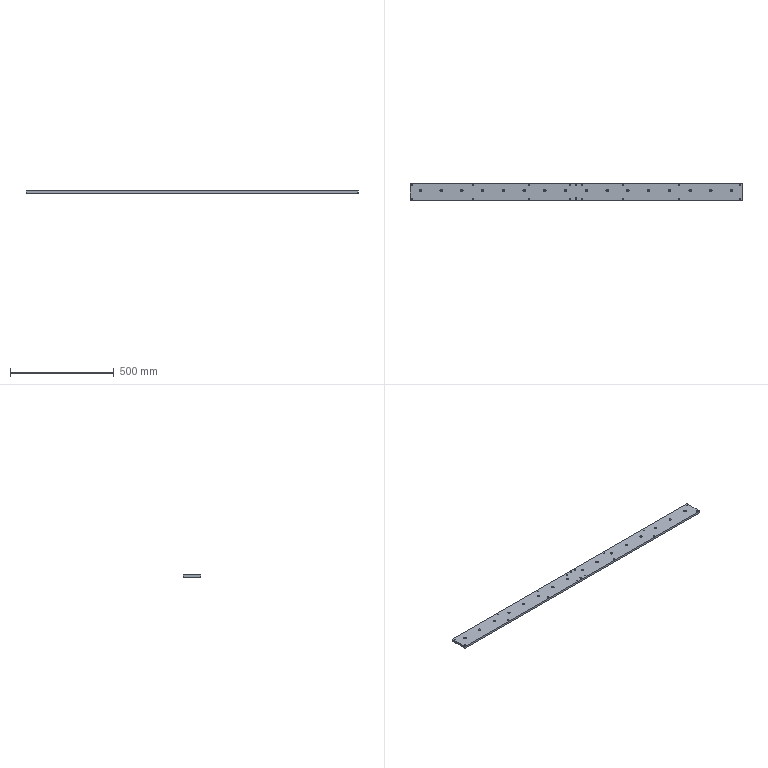CAM job | Mastercam | mm | 8 operations | part box 1600 x 85 x 10
1. Contour (Ramp) | 11 - 12 平铣刀
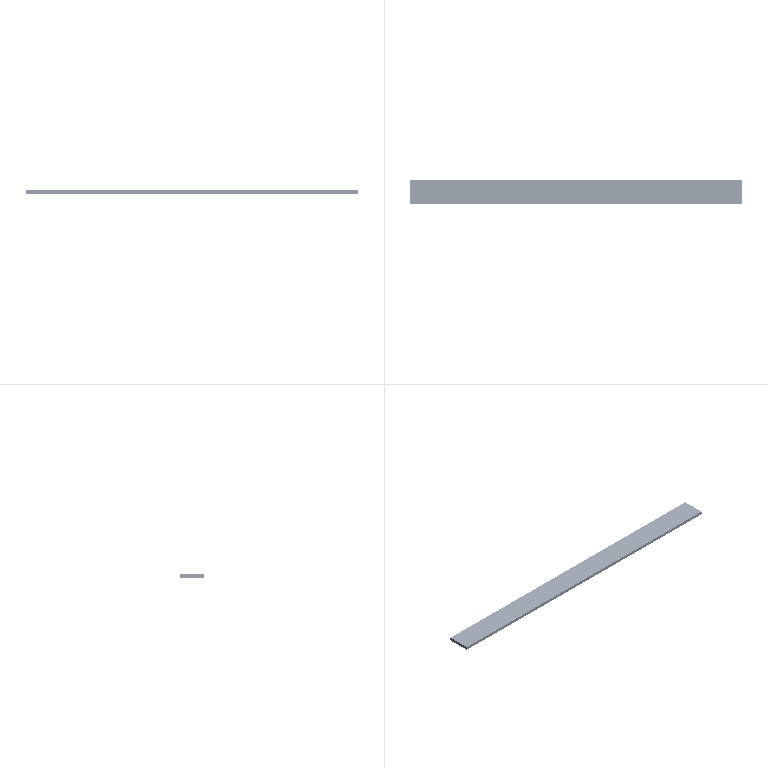2. Contour (2D) | 12 - 12 平铣刀
3. Helix Bore | 6 - 6 平铣刀
4. Drill/Counterbore | 7 - 6 倒角刀
5. Contour (2D chamfer) | 7 - 6 倒角刀
6. Contour (Ramp) | 11 - 12 平铣刀
7. Contour (2D) | 12 - 12 平铣刀
8. Contour (2D chamfer) | 7 - 6 倒角刀